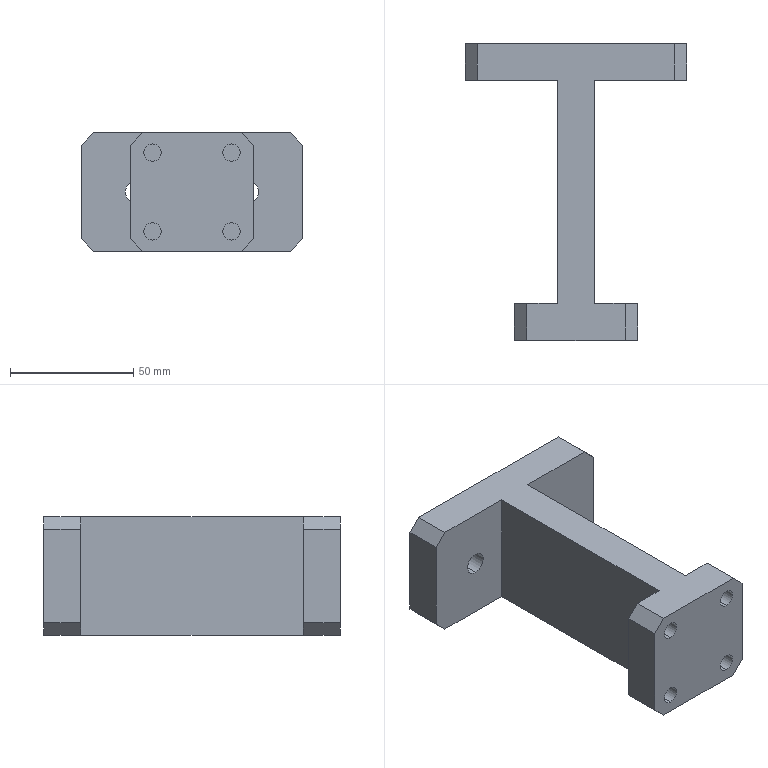Component | SolidWorks | TC020.05-06-2 | 1 solid | 34 faces | box 90 x 120.4 x 48 mm | volume 160170 mm3 | plane 22 | cylinder 12 | commonest cylinder face diameters 7 x8 9 x4 | material Q235A
STEP:
#1=CARTESIAN_POINT('',(4.901,3.307,0.7677));
#2=VERTEX_POINT('',#1);
#3=CARTESIAN_POINT('',(4.901,3.307,0.4921));
#4=VERTEX_POINT('',#3);
#5=CARTESIAN_POINT('',(4.901,3.307,0.6299));
#6=DIRECTION('',(0.,1.,0.));
#7=DIRECTION('',(0.,0.,1.));
#8=AXIS2_PLACEMENT_3D('',#5,#6,#7);
#9=CIRCLE('',#8,0.1378);
#10=EDGE_CURVE('',#2,#4,#9,.T.);
#11=ORIENTED_EDGE('',*,*,#10,.T.);
#12=CARTESIAN_POINT('',(4.901,2.717,0.4921));
#13=VERTEX_POINT('',#12);
#14=CARTESIAN_POINT('',(4.901,4.685,0.4921));
#15=DIRECTION('',(-0.,-1.,0.));
#16=VECTOR('',#15,39.37);
#17=LINE('',#14,#16);
#18=EDGE_CURVE('',#4,#13,#17,.T.);
#19=ORIENTED_EDGE('',*,*,#18,.T.);
#20=CARTESIAN_POINT('',(4.901,2.717,0.7677));
#21=VERTEX_POINT('',#20);
#22=CARTESIAN_POINT('',(4.901,2.717,0.6299));
#23=DIRECTION('',(0.,1.,0.));
#24=DIRECTION('',(0.,0.,-1.));
#25=AXIS2_PLACEMENT_3D('',#22,#23,#24);
#26=CIRCLE('',#25,0.1378);
#27=EDGE_CURVE('',#21,#13,#26,.T.);
#28=ORIENTED_EDGE('',*,*,#27,.F.);
#29=CARTESIAN_POINT('',(4.901,4.685,0.7677));
#30=DIRECTION('',(-0.,-1.,0.));
#31=VECTOR('',#30,39.37);
#32=LINE('',#29,#31);
#33=EDGE_CURVE('',#2,#21,#32,.T.);
#34=ORIENTED_EDGE('',*,*,#33,.F.);
#35=EDGE_LOOP('',(#11,#19,#28,#34));
#36=FACE_OUTER_BOUND('',#35,.T.);
#37=CARTESIAN_POINT('',(4.901,4.685,0.6299));
#38=DIRECTION('',(-0.,-1.,0.));
#39=DIRECTION('',(0.,0.,1.));
#40=AXIS2_PLACEMENT_3D('',#37,#38,#39);
#41=CYLINDRICAL_SURFACE('',#40,0.1378);
#42=ADVANCED_FACE('',(#36),#41,.F.);
#43=CARTESIAN_POINT('',(3.641,3.307,0.7677));
#44=VERTEX_POINT('',#43);
#45=CARTESIAN_POINT('',(3.641,3.307,0.4921));
#46=VERTEX_POINT('',#45);
#47=CARTESIAN_POINT('',(3.641,3.307,0.6299));
#48=DIRECTION('',(0.,1.,0.));
#49=DIRECTION('',(0.,0.,1.));
#50=AXIS2_PLACEMENT_3D('',#47,#48,#49);
#51=CIRCLE('',#50,0.1378);
#52=EDGE_CURVE('',#44,#46,#51,.T.);
#53=ORIENTED_EDGE('',*,*,#52,.T.);
#54=CARTESIAN_POINT('',(3.641,2.717,0.4921));
#55=VERTEX_POINT('',#54);
#56=CARTESIAN_POINT('',(3.641,4.685,0.4921));
#57=DIRECTION('',(-0.,-1.,0.));
#58=VECTOR('',#57,39.37);
#59=LINE('',#56,#58);
#60=EDGE_CURVE('',#46,#55,#59,.T.);
#61=ORIENTED_EDGE('',*,*,#60,.T.);
#62=CARTESIAN_POINT('',(3.641,2.717,0.7677));
#63=VERTEX_POINT('',#62);
#64=CARTESIAN_POINT('',(3.641,2.717,0.6299));
#65=DIRECTION('',(0.,1.,0.));
#66=DIRECTION('',(0.,0.,-1.));
#67=AXIS2_PLACEMENT_3D('',#64,#65,#66);
#68=CIRCLE('',#67,0.1378);
#69=EDGE_CURVE('',#63,#55,#68,.T.);
#70=ORIENTED_EDGE('',*,*,#69,.F.);
#71=CARTESIAN_POINT('',(3.641,4.685,0.7677));
#72=DIRECTION('',(-0.,-1.,0.));
#73=VECTOR('',#72,39.37);
#74=LINE('',#71,#73);
#75=EDGE_CURVE('',#44,#63,#74,.T.);
#76=ORIENTED_EDGE('',*,*,#75,.F.);
#77=EDGE_LOOP('',(#53,#61,#70,#76));
#78=FACE_OUTER_BOUND('',#77,.T.);
#79=CARTESIAN_POINT('',(3.641,4.685,0.6299));
#80=DIRECTION('',(-0.,-1.,0.));
#81=DIRECTION('',(0.,0.,1.));
#82=AXIS2_PLACEMENT_3D('',#79,#80,#81);
#83=CYLINDRICAL_SURFACE('',#82,0.1378);
#84=ADVANCED_FACE('',(#78),#83,.F.);
#85=CARTESIAN_POINT('',(4.901,3.307,-0.4921));
#86=VERTEX_POINT('',#85);
#87=CARTESIAN_POINT('',(4.901,3.307,-0.7677));
#88=VERTEX_POINT('',#87);
#89=CARTESIAN_POINT('',(4.901,3.307,-0.6299));
#90=DIRECTION('',(0.,1.,0.));
#91=DIRECTION('',(0.,0.,1.));
#92=AXIS2_PLACEMENT_3D('',#89,#90,#91);
#93=CIRCLE('',#92,0.1378);
#94=EDGE_CURVE('',#86,#88,#93,.T.);
#95=ORIENTED_EDGE('',*,*,#94,.T.);
#96=CARTESIAN_POINT('',(4.901,2.717,-0.7677));
#97=VERTEX_POINT('',#96);
#98=CARTESIAN_POINT('',(4.901,4.685,-0.7677));
#99=DIRECTION('',(-0.,-1.,0.));
#100=VECTOR('',#99,39.37);
#101=LINE('',#98,#100);
#102=EDGE_CURVE('',#88,#97,#101,.T.);
#103=ORIENTED_EDGE('',*,*,#102,.T.);
#104=CARTESIAN_POINT('',(4.901,2.717,-0.4921));
#105=VERTEX_POINT('',#104);
#106=CARTESIAN_POINT('',(4.901,2.717,-0.6299));
#107=DIRECTION('',(0.,1.,0.));
#108=DIRECTION('',(0.,0.,-1.));
#109=AXIS2_PLACEMENT_3D('',#106,#107,#108);
#110=CIRCLE('',#109,0.1378);
#111=EDGE_CURVE('',#105,#97,#110,.T.);
#112=ORIENTED_EDGE('',*,*,#111,.F.);
#113=CARTESIAN_POINT('',(4.901,4.685,-0.4921));
#114=DIRECTION('',(-0.,-1.,0.));
#115=VECTOR('',#114,39.37);
#116=LINE('',#113,#115);
#117=EDGE_CURVE('',#86,#105,#116,.T.);
#118=ORIENTED_EDGE('',*,*,#117,.F.);
#119=EDGE_LOOP('',(#95,#103,#112,#118));
#120=FACE_OUTER_BOUND('',#119,.T.);
#121=CARTESIAN_POINT('',(4.901,4.685,-0.6299));
#122=DIRECTION('',(-0.,-1.,0.));
#123=DIRECTION('',(0.,0.,1.));
#124=AXIS2_PLACEMENT_3D('',#121,#122,#123);
#125=CYLINDRICAL_SURFACE('',#124,0.1378);
#126=ADVANCED_FACE('',(#120),#125,.F.);
#127=CARTESIAN_POINT('',(3.641,3.307,-0.4921));
#128=VERTEX_POINT('',#127);
#129=CARTESIAN_POINT('',(3.641,3.307,-0.7677));
#130=VERTEX_POINT('',#129);
#131=CARTESIAN_POINT('',(3.641,3.307,-0.6299));
#132=DIRECTION('',(0.,1.,0.));
#133=DIRECTION('',(0.,0.,1.));
#134=AXIS2_PLACEMENT_3D('',#131,#132,#133);
#135=CIRCLE('',#134,0.1378);
#136=EDGE_CURVE('',#128,#130,#135,.T.);
#137=ORIENTED_EDGE('',*,*,#136,.T.);
#138=CARTESIAN_POINT('',(3.641,2.717,-0.7677));
#139=VERTEX_POINT('',#138);
#140=CARTESIAN_POINT('',(3.641,4.685,-0.7677));
#141=DIRECTION('',(-0.,-1.,0.));
#142=VECTOR('',#141,39.37);
#143=LINE('',#140,#142);
#144=EDGE_CURVE('',#130,#139,#143,.T.);
#145=ORIENTED_EDGE('',*,*,#144,.T.);
#146=CARTESIAN_POINT('',(3.641,2.717,-0.4921));
#147=VERTEX_POINT('',#146);
#148=CARTESIAN_POINT('',(3.641,2.717,-0.6299));
#149=DIRECTION('',(0.,1.,0.));
#150=DIRECTION('',(0.,0.,-1.));
#151=AXIS2_PLACEMENT_3D('',#148,#149,#150);
#152=CIRCLE('',#151,0.1378);
#153=EDGE_CURVE('',#147,#139,#152,.T.);
#154=ORIENTED_EDGE('',*,*,#153,.F.);
#155=CARTESIAN_POINT('',(3.641,4.685,-0.4921));
#156=DIRECTION('',(-0.,-1.,0.));
#157=VECTOR('',#156,39.37);
#158=LINE('',#155,#157);
#159=EDGE_CURVE('',#128,#147,#158,.T.);
#160=ORIENTED_EDGE('',*,*,#159,.F.);
#161=EDGE_LOOP('',(#137,#145,#154,#160));
#162=FACE_OUTER_BOUND('',#161,.T.);
#163=CARTESIAN_POINT('',(3.641,4.685,-0.6299));
#164=DIRECTION('',(-0.,-1.,0.));
#165=DIRECTION('',(0.,0.,1.));
#166=AXIS2_PLACEMENT_3D('',#163,#164,#165);
#167=CYLINDRICAL_SURFACE('',#166,0.1378);
#168=ADVANCED_FACE('',(#162),#167,.F.);
#169=CARTESIAN_POINT('',(3.386,6.866,-0.1772));
#170=VERTEX_POINT('',#169);
#171=CARTESIAN_POINT('',(3.386,6.866,0.1772));
#172=VERTEX_POINT('',#171);
#173=CARTESIAN_POINT('',(3.386,6.866,0.));
#174=DIRECTION('',(0.,-1.,0.));
#175=DIRECTION('',(-1.,0.,-0.));
#176=AXIS2_PLACEMENT_3D('',#173,#174,#175);
#177=CIRCLE('',#176,0.1772);
#178=EDGE_CURVE('',#170,#172,#177,.T.);
#179=ORIENTED_EDGE('',*,*,#178,.T.);
#180=CARTESIAN_POINT('',(3.386,7.457,0.1772));
#181=VERTEX_POINT('',#180);
#182=CARTESIAN_POINT('',(3.386,2.716,0.1772));
#183=DIRECTION('',(0.,1.,0.));
#184=VECTOR('',#183,39.37);
#185=LINE('',#182,#184);
#186=EDGE_CURVE('',#172,#181,#185,.T.);
#187=ORIENTED_EDGE('',*,*,#186,.T.);
#188=CARTESIAN_POINT('',(3.386,7.457,-0.1772));
#189=VERTEX_POINT('',#188);
#190=CARTESIAN_POINT('',(3.386,7.457,0.));
#191=DIRECTION('',(0.,1.,0.));
#192=DIRECTION('',(0.,0.,-1.));
#193=AXIS2_PLACEMENT_3D('',#190,#191,#192);
#194=CIRCLE('',#193,0.1772);
#195=EDGE_CURVE('',#181,#189,#194,.T.);
#196=ORIENTED_EDGE('',*,*,#195,.T.);
#197=CARTESIAN_POINT('',(3.386,2.716,-0.1772));
#198=DIRECTION('',(0.,1.,0.));
#199=VECTOR('',#198,39.37);
#200=LINE('',#197,#199);
#201=EDGE_CURVE('',#170,#189,#200,.T.);
#202=ORIENTED_EDGE('',*,*,#201,.F.);
#203=EDGE_LOOP('',(#179,#187,#196,#202));
#204=FACE_OUTER_BOUND('',#203,.T.);
#205=CARTESIAN_POINT('',(3.386,2.716,0.));
#206=DIRECTION('',(0.,1.,0.));
#207=DIRECTION('',(0.,0.,-1.));
#208=AXIS2_PLACEMENT_3D('',#205,#206,#207);
#209=CYLINDRICAL_SURFACE('',#208,0.1772);
#210=ADVANCED_FACE('',(#204),#209,.F.);
#211=CARTESIAN_POINT('',(5.157,6.866,-0.1772));
#212=VERTEX_POINT('',#211);
#213=CARTESIAN_POINT('',(5.157,6.866,0.1772));
#214=VERTEX_POINT('',#213);
#215=CARTESIAN_POINT('',(5.157,6.866,0.));
#216=DIRECTION('',(-0.,-1.,-0.));
#217=DIRECTION('',(-1.,0.,-0.));
#218=AXIS2_PLACEMENT_3D('',#215,#216,#217);
#219=CIRCLE('',#218,0.1772);
#220=EDGE_CURVE('',#212,#214,#219,.T.);
#221=ORIENTED_EDGE('',*,*,#220,.T.);
#222=CARTESIAN_POINT('',(5.157,7.457,0.1772));
#223=VERTEX_POINT('',#222);
#224=CARTESIAN_POINT('',(5.157,2.716,0.1772));
#225=DIRECTION('',(0.,1.,0.));
#226=VECTOR('',#225,39.37);
#227=LINE('',#224,#226);
#228=EDGE_CURVE('',#214,#223,#227,.T.);
#229=ORIENTED_EDGE('',*,*,#228,.T.);
#230=CARTESIAN_POINT('',(5.157,7.457,-0.1772));
#231=VERTEX_POINT('',#230);
#232=CARTESIAN_POINT('',(5.157,7.457,0.));
#233=DIRECTION('',(0.,1.,0.));
#234=DIRECTION('',(0.,0.,-1.));
#235=AXIS2_PLACEMENT_3D('',#232,#233,#234);
#236=CIRCLE('',#235,0.1772);
#237=EDGE_CURVE('',#223,#231,#236,.T.);
#238=ORIENTED_EDGE('',*,*,#237,.T.);
#239=CARTESIAN_POINT('',(5.157,2.716,-0.1772));
#240=DIRECTION('',(0.,1.,0.));
#241=VECTOR('',#240,39.37);
#242=LINE('',#239,#241);
#243=EDGE_CURVE('',#212,#231,#242,.T.);
#244=ORIENTED_EDGE('',*,*,#243,.F.);
#245=EDGE_LOOP('',(#221,#229,#238,#244));
#246=FACE_OUTER_BOUND('',#245,.T.);
#247=CARTESIAN_POINT('',(5.157,2.716,0.));
#248=DIRECTION('',(0.,1.,0.));
#249=DIRECTION('',(0.,0.,-1.));
#250=AXIS2_PLACEMENT_3D('',#247,#248,#249);
#251=CYLINDRICAL_SURFACE('',#250,0.1772);
#252=ADVANCED_FACE('',(#246),#251,.F.);
#253=CARTESIAN_POINT('',(3.484,2.717,0.9449));
#254=VERTEX_POINT('',#253);
#255=CARTESIAN_POINT('',(5.059,2.717,0.9449));
#256=VERTEX_POINT('',#255);
#257=CARTESIAN_POINT('',(3.287,2.717,0.9449));
#258=DIRECTION('',(1.,-0.,0.));
#259=VECTOR('',#258,39.37);
#260=LINE('',#257,#259);
#261=EDGE_CURVE('',#254,#256,#260,.T.);
#262=ORIENTED_EDGE('',*,*,#261,.F.);
#263=CARTESIAN_POINT('',(3.287,2.717,0.748));
#264=VERTEX_POINT('',#263);
#265=CARTESIAN_POINT('',(3.484,2.717,0.9449));
#266=DIRECTION('',(-0.7071,0.,-0.7071));
#267=VECTOR('',#266,39.37);
#268=LINE('',#265,#267);
#269=EDGE_CURVE('',#254,#264,#268,.T.);
#270=ORIENTED_EDGE('',*,*,#269,.T.);
#271=CARTESIAN_POINT('',(3.287,2.717,-0.748));
#272=VERTEX_POINT('',#271);
#273=CARTESIAN_POINT('',(3.287,2.717,0.9449));
#274=DIRECTION('',(0.,0.,-1.));
#275=VECTOR('',#274,39.37);
#276=LINE('',#273,#275);
#277=EDGE_CURVE('',#264,#272,#276,.T.);
#278=ORIENTED_EDGE('',*,*,#277,.T.);
#279=CARTESIAN_POINT('',(3.484,2.717,-0.9449));
#280=VERTEX_POINT('',#279);
#281=CARTESIAN_POINT('',(3.287,2.717,-0.748));
#282=DIRECTION('',(0.7071,-0.,-0.7071));
#283=VECTOR('',#282,39.37);
#284=LINE('',#281,#283);
#285=EDGE_CURVE('',#272,#280,#284,.T.);
#286=ORIENTED_EDGE('',*,*,#285,.T.);
#287=CARTESIAN_POINT('',(5.059,2.717,-0.9449));
#288=VERTEX_POINT('',#287);
#289=CARTESIAN_POINT('',(3.287,2.717,-0.9449));
#290=DIRECTION('',(1.,-0.,0.));
#291=VECTOR('',#290,39.37);
#292=LINE('',#289,#291);
#293=EDGE_CURVE('',#280,#288,#292,.T.);
#294=ORIENTED_EDGE('',*,*,#293,.T.);
#295=CARTESIAN_POINT('',(5.256,2.717,-0.748));
#296=VERTEX_POINT('',#295);
#297=CARTESIAN_POINT('',(5.256,2.717,-0.748));
#298=DIRECTION('',(0.7071,-0.,0.7071));
#299=VECTOR('',#298,39.37);
#300=LINE('',#297,#299);
#301=EDGE_CURVE('',#288,#296,#300,.T.);
#302=ORIENTED_EDGE('',*,*,#301,.T.);
#303=CARTESIAN_POINT('',(5.256,2.717,0.748));
#304=VERTEX_POINT('',#303);
#305=CARTESIAN_POINT('',(5.256,2.717,0.9449));
#306=DIRECTION('',(0.,0.,-1.));
#307=VECTOR('',#306,39.37);
#308=LINE('',#305,#307);
#309=EDGE_CURVE('',#304,#296,#308,.T.);
#310=ORIENTED_EDGE('',*,*,#309,.F.);
#311=CARTESIAN_POINT('',(5.059,2.717,0.9449));
#312=DIRECTION('',(-0.7071,0.,0.7071));
#313=VECTOR('',#312,39.37);
#314=LINE('',#311,#313);
#315=EDGE_CURVE('',#304,#256,#314,.T.);
#316=ORIENTED_EDGE('',*,*,#315,.T.);
#317=EDGE_LOOP('',(#262,#270,#278,#286,#294,#302,#310,#316));
#318=FACE_OUTER_BOUND('',#317,.T.);
#319=ORIENTED_EDGE('',*,*,#153,.T.);
#320=CARTESIAN_POINT('',(3.641,2.717,-0.6299));
#321=DIRECTION('',(0.,1.,0.));
#322=DIRECTION('',(0.,0.,-1.));
#323=AXIS2_PLACEMENT_3D('',#320,#321,#322);
#324=CIRCLE('',#323,0.1378);
#325=EDGE_CURVE('',#139,#147,#324,.T.);
#326=ORIENTED_EDGE('',*,*,#325,.T.);
#327=EDGE_LOOP('',(#319,#326));
#328=FACE_BOUND('',#327,.T.);
#329=ORIENTED_EDGE('',*,*,#111,.T.);
#330=CARTESIAN_POINT('',(4.901,2.717,-0.6299));
#331=DIRECTION('',(0.,1.,0.));
#332=DIRECTION('',(0.,0.,-1.));
#333=AXIS2_PLACEMENT_3D('',#330,#331,#332);
#334=CIRCLE('',#333,0.1378);
#335=EDGE_CURVE('',#97,#105,#334,.T.);
#336=ORIENTED_EDGE('',*,*,#335,.T.);
#337=EDGE_LOOP('',(#329,#336));
#338=FACE_BOUND('',#337,.T.);
#339=ORIENTED_EDGE('',*,*,#69,.T.);
#340=CARTESIAN_POINT('',(3.641,2.717,0.6299));
#341=DIRECTION('',(0.,1.,0.));
#342=DIRECTION('',(0.,0.,-1.));
#343=AXIS2_PLACEMENT_3D('',#340,#341,#342);
#344=CIRCLE('',#343,0.1378);
#345=EDGE_CURVE('',#55,#63,#344,.T.);
#346=ORIENTED_EDGE('',*,*,#345,.T.);
#347=EDGE_LOOP('',(#339,#346));
#348=FACE_BOUND('',#347,.T.);
#349=ORIENTED_EDGE('',*,*,#27,.T.);
#350=CARTESIAN_POINT('',(4.901,2.717,0.6299));
#351=DIRECTION('',(0.,1.,0.));
#352=DIRECTION('',(0.,0.,-1.));
#353=AXIS2_PLACEMENT_3D('',#350,#351,#352);
#354=CIRCLE('',#353,0.1378);
#355=EDGE_CURVE('',#13,#21,#354,.T.);
#356=ORIENTED_EDGE('',*,*,#355,.T.);
#357=EDGE_LOOP('',(#349,#356));
#358=FACE_BOUND('',#357,.T.);
#359=CARTESIAN_POINT('',(3.287,2.717,0.9449));
#360=DIRECTION('',(0.,1.,0.));
#361=DIRECTION('',(0.,0.,-1.));
#362=AXIS2_PLACEMENT_3D('',#359,#360,#361);
#363=PLANE('',#362);
#364=ADVANCED_FACE('',(#318,#328,#338,#348,#358),#363,.F.);
#365=CARTESIAN_POINT('',(5.059,3.307,0.9449));
#366=VERTEX_POINT('',#365);
#367=CARTESIAN_POINT('',(4.567,3.307,0.9449));
#368=VERTEX_POINT('',#367);
#369=CARTESIAN_POINT('',(4.567,3.307,0.9449));
#370=DIRECTION('',(-1.,0.,-0.));
#371=VECTOR('',#370,39.37);
#372=LINE('',#369,#371);
#373=EDGE_CURVE('',#366,#368,#372,.T.);
#374=ORIENTED_EDGE('',*,*,#373,.F.);
#375=CARTESIAN_POINT('',(5.256,3.307,0.748));
#376=VERTEX_POINT('',#375);
#377=CARTESIAN_POINT('',(5.059,3.307,0.9449));
#378=DIRECTION('',(0.7071,-0.,-0.7071));
#379=VECTOR('',#378,39.37);
#380=LINE('',#377,#379);
#381=EDGE_CURVE('',#366,#376,#380,.T.);
#382=ORIENTED_EDGE('',*,*,#381,.T.);
#383=CARTESIAN_POINT('',(5.256,3.307,-0.748));
#384=VERTEX_POINT('',#383);
#385=CARTESIAN_POINT('',(5.256,3.307,0.9449));
#386=DIRECTION('',(0.,0.,-1.));
#387=VECTOR('',#386,39.37);
#388=LINE('',#385,#387);
#389=EDGE_CURVE('',#376,#384,#388,.T.);
#390=ORIENTED_EDGE('',*,*,#389,.T.);
#391=CARTESIAN_POINT('',(5.059,3.307,-0.9449));
#392=VERTEX_POINT('',#391);
#393=CARTESIAN_POINT('',(5.256,3.307,-0.748));
#394=DIRECTION('',(-0.7071,0.,-0.7071));
#395=VECTOR('',#394,39.37);
#396=LINE('',#393,#395);
#397=EDGE_CURVE('',#384,#392,#396,.T.);
#398=ORIENTED_EDGE('',*,*,#397,.T.);
#399=CARTESIAN_POINT('',(4.567,3.307,-0.9449));
#400=VERTEX_POINT('',#399);
#401=CARTESIAN_POINT('',(4.567,3.307,-0.9449));
#402=DIRECTION('',(-1.,0.,-0.));
#403=VECTOR('',#402,39.37);
#404=LINE('',#401,#403);
#405=EDGE_CURVE('',#392,#400,#404,.T.);
#406=ORIENTED_EDGE('',*,*,#405,.T.);
#407=CARTESIAN_POINT('',(4.567,3.307,0.9449));
#408=DIRECTION('',(0.,0.,-1.));
#409=VECTOR('',#408,39.37);
#410=LINE('',#407,#409);
#411=EDGE_CURVE('',#368,#400,#410,.T.);
#412=ORIENTED_EDGE('',*,*,#411,.F.);
#413=EDGE_LOOP('',(#374,#382,#390,#398,#406,#412));
#414=FACE_OUTER_BOUND('',#413,.T.);
#415=ORIENTED_EDGE('',*,*,#94,.F.);
#416=CARTESIAN_POINT('',(4.901,3.307,-0.6299));
#417=DIRECTION('',(0.,1.,0.));
#418=DIRECTION('',(0.,0.,1.));
#419=AXIS2_PLACEMENT_3D('',#416,#417,#418);
#420=CIRCLE('',#419,0.1378);
#421=EDGE_CURVE('',#88,#86,#420,.T.);
#422=ORIENTED_EDGE('',*,*,#421,.F.);
#423=EDGE_LOOP('',(#415,#422));
#424=FACE_BOUND('',#423,.T.);
#425=ORIENTED_EDGE('',*,*,#10,.F.);
#426=CARTESIAN_POINT('',(4.901,3.307,0.6299));
#427=DIRECTION('',(0.,1.,0.));
#428=DIRECTION('',(0.,0.,1.));
#429=AXIS2_PLACEMENT_3D('',#426,#427,#428);
#430=CIRCLE('',#429,0.1378);
#431=EDGE_CURVE('',#4,#2,#430,.T.);
#432=ORIENTED_EDGE('',*,*,#431,.F.);
#433=EDGE_LOOP('',(#425,#432));
#434=FACE_BOUND('',#433,.T.);
#435=CARTESIAN_POINT('',(4.567,3.307,0.9449));
#436=DIRECTION('',(-0.,-1.,-0.));
#437=DIRECTION('',(-0.,0.,1.));
#438=AXIS2_PLACEMENT_3D('',#435,#436,#437);
#439=PLANE('',#438);
#440=ADVANCED_FACE('',(#414,#424,#434),#439,.F.);
#441=CARTESIAN_POINT('',(3.287,3.307,0.748));
#442=VERTEX_POINT('',#441);
#443=CARTESIAN_POINT('',(3.287,3.307,-0.748));
#444=VERTEX_POINT('',#443);
#445=CARTESIAN_POINT('',(3.287,3.307,0.9449));
#446=DIRECTION('',(0.,0.,-1.));
#447=VECTOR('',#446,39.37);
#448=LINE('',#445,#447);
#449=EDGE_CURVE('',#442,#444,#448,.T.);
#450=ORIENTED_EDGE('',*,*,#449,.F.);
#451=CARTESIAN_POINT('',(3.484,3.307,0.9449));
#452=VERTEX_POINT('',#451);
#453=CARTESIAN_POINT('',(3.484,3.307,0.9449));
#454=DIRECTION('',(0.7071,-0.,0.7071));
#455=VECTOR('',#454,39.37);
#456=LINE('',#453,#455);
#457=EDGE_CURVE('',#442,#452,#456,.T.);
#458=ORIENTED_EDGE('',*,*,#457,.T.);
#459=CARTESIAN_POINT('',(3.976,3.307,0.9449));
#460=VERTEX_POINT('',#459);
#461=CARTESIAN_POINT('',(3.976,3.307,0.9449));
#462=DIRECTION('',(-1.,0.,-0.));
#463=VECTOR('',#462,39.37);
#464=LINE('',#461,#463);
#465=EDGE_CURVE('',#460,#452,#464,.T.);
#466=ORIENTED_EDGE('',*,*,#465,.F.);
#467=CARTESIAN_POINT('',(3.976,3.307,-0.9449));
#468=VERTEX_POINT('',#467);
#469=CARTESIAN_POINT('',(3.976,3.307,0.9449));
#470=DIRECTION('',(0.,0.,-1.));
#471=VECTOR('',#470,39.37);
#472=LINE('',#469,#471);
#473=EDGE_CURVE('',#460,#468,#472,.T.);
#474=ORIENTED_EDGE('',*,*,#473,.T.);
#475=CARTESIAN_POINT('',(3.484,3.307,-0.9449));
#476=VERTEX_POINT('',#475);
#477=CARTESIAN_POINT('',(3.976,3.307,-0.9449));
#478=DIRECTION('',(-1.,0.,-0.));
#479=VECTOR('',#478,39.37);
#480=LINE('',#477,#479);
#481=EDGE_CURVE('',#468,#476,#480,.T.);
#482=ORIENTED_EDGE('',*,*,#481,.T.);
#483=CARTESIAN_POINT('',(3.287,3.307,-0.748));
#484=DIRECTION('',(-0.7071,0.,0.7071));
#485=VECTOR('',#484,39.37);
#486=LINE('',#483,#485);
#487=EDGE_CURVE('',#476,#444,#486,.T.);
#488=ORIENTED_EDGE('',*,*,#487,.T.);
#489=EDGE_LOOP('',(#450,#458,#466,#474,#482,#488));
#490=FACE_OUTER_BOUND('',#489,.T.);
#491=ORIENTED_EDGE('',*,*,#136,.F.);
#492=CARTESIAN_POINT('',(3.641,3.307,-0.6299));
#493=DIRECTION('',(0.,1.,0.));
#494=DIRECTION('',(0.,0.,1.));
#495=AXIS2_PLACEMENT_3D('',#492,#493,#494);
#496=CIRCLE('',#495,0.1378);
#497=EDGE_CURVE('',#130,#128,#496,.T.);
#498=ORIENTED_EDGE('',*,*,#497,.F.);
#499=EDGE_LOOP('',(#491,#498));
#500=FACE_BOUND('',#499,.T.);
#501=ORIENTED_EDGE('',*,*,#52,.F.);
#502=CARTESIAN_POINT('',(3.641,3.307,0.6299));
#503=DIRECTION('',(0.,1.,0.));
#504=DIRECTION('',(0.,0.,1.));
#505=AXIS2_PLACEMENT_3D('',#502,#503,#504);
#506=CIRCLE('',#505,0.1378);
#507=EDGE_CURVE('',#46,#44,#506,.T.);
#508=ORIENTED_EDGE('',*,*,#507,.F.);
#509=EDGE_LOOP('',(#501,#508));
#510=FACE_BOUND('',#509,.T.);
#511=CARTESIAN_POINT('',(3.976,3.307,0.9449));
#512=DIRECTION('',(-0.,-1.,-0.));
#513=DIRECTION('',(-0.,0.,1.));
#514=AXIS2_PLACEMENT_3D('',#511,#512,#513);
#515=PLANE('',#514);
#516=ADVANCED_FACE('',(#490,#500,#510),#515,.F.);
#517=ORIENTED_EDGE('',*,*,#178,.F.);
#518=CARTESIAN_POINT('',(3.386,6.866,0.));
#519=DIRECTION('',(0.,-1.,0.));
#520=DIRECTION('',(-1.,0.,-0.));
#521=AXIS2_PLACEMENT_3D('',#518,#519,#520);
#522=CIRCLE('',#521,0.1772);
#523=EDGE_CURVE('',#172,#170,#522,.T.);
#524=ORIENTED_EDGE('',*,*,#523,.F.);
#525=EDGE_LOOP('',(#517,#524));
#526=FACE_BOUND('',#525,.T.);
#527=CARTESIAN_POINT('',(2.697,6.866,0.9449));
#528=VERTEX_POINT('',#527);
#529=CARTESIAN_POINT('',(3.976,6.866,0.9449));
#530=VERTEX_POINT('',#529);
#531=CARTESIAN_POINT('',(2.5,6.866,0.9449));
#532=DIRECTION('',(1.,0.,0.));
#533=VECTOR('',#532,39.37);
#534=LINE('',#531,#533);
#535=EDGE_CURVE('',#528,#530,#534,.T.);
#536=ORIENTED_EDGE('',*,*,#535,.F.);
#537=CARTESIAN_POINT('',(2.5,6.866,0.748));
#538=VERTEX_POINT('',#537);
#539=CARTESIAN_POINT('',(2.697,6.866,0.9449));
#540=DIRECTION('',(-0.7071,-0.,-0.7071));
#541=VECTOR('',#540,39.37);
#542=LINE('',#539,#541);
#543=EDGE_CURVE('',#528,#538,#542,.T.);
#544=ORIENTED_EDGE('',*,*,#543,.T.);
#545=CARTESIAN_POINT('',(2.5,6.866,-0.748));
#546=VERTEX_POINT('',#545);
#547=CARTESIAN_POINT('',(2.5,6.866,0.9449));
#548=DIRECTION('',(0.,0.,-1.));
#549=VECTOR('',#548,39.37);
#550=LINE('',#547,#549);
#551=EDGE_CURVE('',#538,#546,#550,.T.);
#552=ORIENTED_EDGE('',*,*,#551,.T.);
#553=CARTESIAN_POINT('',(2.697,6.866,-0.9449));
#554=VERTEX_POINT('',#553);
#555=CARTESIAN_POINT('',(2.5,6.866,-0.748));
#556=DIRECTION('',(0.7071,0.,-0.7071));
#557=VECTOR('',#556,39.37);
#558=LINE('',#555,#557);
#559=EDGE_CURVE('',#546,#554,#558,.T.);
#560=ORIENTED_EDGE('',*,*,#559,.T.);
#561=CARTESIAN_POINT('',(3.976,6.866,-0.9449));
#562=VERTEX_POINT('',#561);
#563=CARTESIAN_POINT('',(2.5,6.866,-0.9449));
#564=DIRECTION('',(1.,0.,0.));
#565=VECTOR('',#564,39.37);
#566=LINE('',#563,#565);
#567=EDGE_CURVE('',#554,#562,#566,.T.);
#568=ORIENTED_EDGE('',*,*,#567,.T.);
#569=CARTESIAN_POINT('',(3.976,6.866,0.9449));
#570=DIRECTION('',(0.,0.,-1.));
#571=VECTOR('',#570,39.37);
#572=LINE('',#569,#571);
#573=EDGE_CURVE('',#530,#562,#572,.T.);
#574=ORIENTED_EDGE('',*,*,#573,.F.);
#575=EDGE_LOOP('',(#536,#544,#552,#560,#568,#574));
#576=FACE_OUTER_BOUND('',#575,.T.);
#577=CARTESIAN_POINT('',(2.5,6.866,0.9449));
#578=DIRECTION('',(-0.,1.,-0.));
#579=DIRECTION('',(-1.,-0.,-0.));
#580=AXIS2_PLACEMENT_3D('',#577,#578,#579);
#581=PLANE('',#580);
#582=ADVANCED_FACE('',(#526,#576),#581,.F.);
#583=CARTESIAN_POINT('',(3.976,6.866,-0.9449));
#584=DIRECTION('',(-0.,-1.,0.));
#585=VECTOR('',#584,39.37);
#586=LINE('',#583,#585);
#587=EDGE_CURVE('',#562,#468,#586,.T.);
#588=ORIENTED_EDGE('',*,*,#587,.T.);
#589=ORIENTED_EDGE('',*,*,#473,.F.);
#590=CARTESIAN_POINT('',(3.976,6.866,0.9449));
#591=DIRECTION('',(-0.,-1.,0.));
#592=VECTOR('',#591,39.37);
#593=LINE('',#590,#592);
#594=EDGE_CURVE('',#530,#460,#593,.T.);
#595=ORIENTED_EDGE('',*,*,#594,.F.);
#596=ORIENTED_EDGE('',*,*,#573,.T.);
#597=EDGE_LOOP('',(#588,#589,#595,#596));
#598=FACE_OUTER_BOUND('',#597,.T.);
#599=CARTESIAN_POINT('',(3.976,6.866,0.9449));
#600=DIRECTION('',(1.,-0.,0.));
#601=DIRECTION('',(-0.,0.,1.));
#602=AXIS2_PLACEMENT_3D('',#599,#600,#601);
#603=PLANE('',#602);
#604=ADVANCED_FACE('',(#598),#603,.F.);
#605=ORIENTED_EDGE('',*,*,#277,.F.);
#606=CARTESIAN_POINT('',(3.287,3.307,0.748));
#607=DIRECTION('',(0.,1.,0.));
#608=VECTOR('',#607,39.37);
#609=LINE('',#606,#608);
#610=EDGE_CURVE('',#264,#442,#609,.T.);
#611=ORIENTED_EDGE('',*,*,#610,.T.);
#612=ORIENTED_EDGE('',*,*,#449,.T.);
#613=CARTESIAN_POINT('',(3.287,2.717,-0.748));
#614=DIRECTION('',(-0.,-1.,0.));
#615=VECTOR('',#614,39.37);
#616=LINE('',#613,#615);
#617=EDGE_CURVE('',#444,#272,#616,.T.);
#618=ORIENTED_EDGE('',*,*,#617,.T.);
#619=EDGE_LOOP('',(#605,#611,#612,#618));
#620=FACE_OUTER_BOUND('',#619,.T.);
#621=CARTESIAN_POINT('',(3.287,3.307,0.9449));
#622=DIRECTION('',(1.,-0.,0.));
#623=DIRECTION('',(-0.,0.,1.));
#624=AXIS2_PLACEMENT_3D('',#621,#622,#623);
#625=PLANE('',#624);
#626=ADVANCED_FACE('',(#620),#625,.F.);
#627=ORIENTED_EDGE('',*,*,#389,.F.);
#628=CARTESIAN_POINT('',(5.256,3.307,0.748));
#629=DIRECTION('',(-0.,-1.,0.));
#630=VECTOR('',#629,39.37);
#631=LINE('',#628,#630);
#632=EDGE_CURVE('',#376,#304,#631,.T.);
#633=ORIENTED_EDGE('',*,*,#632,.T.);
#634=ORIENTED_EDGE('',*,*,#309,.T.);
#635=CARTESIAN_POINT('',(5.256,3.307,-0.748));
#636=DIRECTION('',(0.,1.,0.));
#637=VECTOR('',#636,39.37);
#638=LINE('',#635,#637);
#639=EDGE_CURVE('',#296,#384,#638,.T.);
#640=ORIENTED_EDGE('',*,*,#639,.T.);
#641=EDGE_LOOP('',(#627,#633,#634,#640));
#642=FACE_OUTER_BOUND('',#641,.T.);
#643=CARTESIAN_POINT('',(5.256,3.307,0.9449));
#644=DIRECTION('',(-1.,0.,-0.));
#645=DIRECTION('',(0.,0.,-1.));
#646=AXIS2_PLACEMENT_3D('',#643,#644,#645);
#647=PLANE('',#646);
#648=ADVANCED_FACE('',(#642),#647,.F.);
#649=CARTESIAN_POINT('',(4.567,6.866,-0.9449));
#650=VERTEX_POINT('',#649);
#651=CARTESIAN_POINT('',(4.567,6.866,-0.9449));
#652=DIRECTION('',(0.,1.,0.));
#653=VECTOR('',#652,39.37);
#654=LINE('',#651,#653);
#655=EDGE_CURVE('',#400,#650,#654,.T.);
#656=ORIENTED_EDGE('',*,*,#655,.T.);
#657=CARTESIAN_POINT('',(4.567,6.866,0.9449));
#658=VERTEX_POINT('',#657);
#659=CARTESIAN_POINT('',(4.567,6.866,0.9449));
#660=DIRECTION('',(0.,0.,-1.));
#661=VECTOR('',#660,39.37);
#662=LINE('',#659,#661);
#663=EDGE_CURVE('',#658,#650,#662,.T.);
#664=ORIENTED_EDGE('',*,*,#663,.F.);
#665=CARTESIAN_POINT('',(4.567,6.866,0.9449));
#666=DIRECTION('',(0.,1.,0.));
#667=VECTOR('',#666,39.37);
#668=LINE('',#665,#667);
#669=EDGE_CURVE('',#368,#658,#668,.T.);
#670=ORIENTED_EDGE('',*,*,#669,.F.);
#671=ORIENTED_EDGE('',*,*,#411,.T.);
#672=EDGE_LOOP('',(#656,#664,#670,#671));
#673=FACE_OUTER_BOUND('',#672,.T.);
#674=CARTESIAN_POINT('',(4.567,6.866,0.9449));
#675=DIRECTION('',(-1.,0.,-0.));
#676=DIRECTION('',(0.,0.,-1.));
#677=AXIS2_PLACEMENT_3D('',#674,#675,#676);
#678=PLANE('',#677);
#679=ADVANCED_FACE('',(#673),#678,.F.);
#680=ORIENTED_EDGE('',*,*,#220,.F.);
#681=CARTESIAN_POINT('',(5.157,6.866,0.));
#682=DIRECTION('',(-0.,-1.,-0.));
#683=DIRECTION('',(-1.,0.,-0.));
#684=AXIS2_PLACEMENT_3D('',#681,#682,#683);
#685=CIRCLE('',#684,0.1772);
#686=EDGE_CURVE('',#214,#212,#685,.T.);
#687=ORIENTED_EDGE('',*,*,#686,.F.);
#688=EDGE_LOOP('',(#680,#687));
#689=FACE_BOUND('',#688,.T.);
#690=CARTESIAN_POINT('',(6.043,6.866,0.748));
#691=VERTEX_POINT('',#690);
#692=CARTESIAN_POINT('',(6.043,6.866,-0.748));
#693=VERTEX_POINT('',#692);
#694=CARTESIAN_POINT('',(6.043,6.866,0.9449));
#695=DIRECTION('',(0.,0.,-1.));
#696=VECTOR('',#695,39.37);
#697=LINE('',#694,#696);
#698=EDGE_CURVE('',#691,#693,#697,.T.);
#699=ORIENTED_EDGE('',*,*,#698,.F.);
#700=CARTESIAN_POINT('',(5.846,6.866,0.9449));
#701=VERTEX_POINT('',#700);
#702=CARTESIAN_POINT('',(5.846,6.866,0.9449));
#703=DIRECTION('',(-0.7071,0.,0.7071));
#704=VECTOR('',#703,39.37);
#705=LINE('',#702,#704);
#706=EDGE_CURVE('',#691,#701,#705,.T.);
#707=ORIENTED_EDGE('',*,*,#706,.T.);
#708=CARTESIAN_POINT('',(6.043,6.866,0.9449));
#709=DIRECTION('',(1.,-0.,0.));
#710=VECTOR('',#709,39.37);
#711=LINE('',#708,#710);
#712=EDGE_CURVE('',#658,#701,#711,.T.);
#713=ORIENTED_EDGE('',*,*,#712,.F.);
#714=ORIENTED_EDGE('',*,*,#663,.T.);
#715=CARTESIAN_POINT('',(5.846,6.866,-0.9449));
#716=VERTEX_POINT('',#715);
#717=CARTESIAN_POINT('',(6.043,6.866,-0.9449));
#718=DIRECTION('',(1.,-0.,0.));
#719=VECTOR('',#718,39.37);
#720=LINE('',#717,#719);
#721=EDGE_CURVE('',#650,#716,#720,.T.);
#722=ORIENTED_EDGE('',*,*,#721,.T.);
#723=CARTESIAN_POINT('',(6.043,6.866,-0.748));
#724=DIRECTION('',(0.7071,-0.,0.7071));
#725=VECTOR('',#724,39.37);
#726=LINE('',#723,#725);
#727=EDGE_CURVE('',#716,#693,#726,.T.);
#728=ORIENTED_EDGE('',*,*,#727,.T.);
#729=EDGE_LOOP('',(#699,#707,#713,#714,#722,#728));
#730=FACE_OUTER_BOUND('',#729,.T.);
#731=CARTESIAN_POINT('',(6.043,6.866,0.9449));
#732=DIRECTION('',(0.,1.,0.));
#733=DIRECTION('',(-1.,0.,-0.));
#734=AXIS2_PLACEMENT_3D('',#731,#732,#733);
#735=PLANE('',#734);
#736=ADVANCED_FACE('',(#689,#730),#735,.F.);
#737=CARTESIAN_POINT('',(6.043,7.457,0.748));
#738=VERTEX_POINT('',#737);
#739=CARTESIAN_POINT('',(6.043,7.457,-0.748));
#740=VERTEX_POINT('',#739);
#741=CARTESIAN_POINT('',(6.043,7.457,0.9449));
#742=DIRECTION('',(0.,0.,-1.));
#743=VECTOR('',#742,39.37);
#744=LINE('',#741,#743);
#745=EDGE_CURVE('',#738,#740,#744,.T.);
#746=ORIENTED_EDGE('',*,*,#745,.F.);
#747=CARTESIAN_POINT('',(6.043,7.457,0.748));
#748=DIRECTION('',(-0.,-1.,0.));
#749=VECTOR('',#748,39.37);
#750=LINE('',#747,#749);
#751=EDGE_CURVE('',#738,#691,#750,.T.);
#752=ORIENTED_EDGE('',*,*,#751,.T.);
#753=ORIENTED_EDGE('',*,*,#698,.T.);
#754=CARTESIAN_POINT('',(6.043,7.457,-0.748));
#755=DIRECTION('',(0.,1.,0.));
#756=VECTOR('',#755,39.37);
#757=LINE('',#754,#756);
#758=EDGE_CURVE('',#693,#740,#757,.T.);
#759=ORIENTED_EDGE('',*,*,#758,.T.);
#760=EDGE_LOOP('',(#746,#752,#753,#759));
#761=FACE_OUTER_BOUND('',#760,.T.);
#762=CARTESIAN_POINT('',(6.043,7.457,0.9449));
#763=DIRECTION('',(-1.,0.,-0.));
#764=DIRECTION('',(0.,0.,-1.));
#765=AXIS2_PLACEMENT_3D('',#762,#763,#764);
#766=PLANE('',#765);
#767=ADVANCED_FACE('',(#761),#766,.F.);
#768=CARTESIAN_POINT('',(3.386,7.457,0.));
#769=DIRECTION('',(0.,1.,0.));
#770=DIRECTION('',(0.,0.,-1.));
#771=AXIS2_PLACEMENT_3D('',#768,#769,#770);
#772=CIRCLE('',#771,0.1772);
#773=EDGE_CURVE('',#189,#181,#772,.T.);
#774=ORIENTED_EDGE('',*,*,#773,.F.);
#775=ORIENTED_EDGE('',*,*,#195,.F.);
#776=EDGE_LOOP('',(#774,#775));
#777=FACE_BOUND('',#776,.T.);
#778=CARTESIAN_POINT('',(5.157,7.457,0.));
#779=DIRECTION('',(0.,1.,0.));
#780=DIRECTION('',(0.,0.,-1.));
#781=AXIS2_PLACEMENT_3D('',#778,#779,#780);
#782=CIRCLE('',#781,0.1772);
#783=EDGE_CURVE('',#231,#223,#782,.T.);
#784=ORIENTED_EDGE('',*,*,#783,.F.);
#785=ORIENTED_EDGE('',*,*,#237,.F.);
#786=EDGE_LOOP('',(#784,#785));
#787=FACE_BOUND('',#786,.T.);
#788=CARTESIAN_POINT('',(5.846,7.457,0.9449));
#789=VERTEX_POINT('',#788);
#790=CARTESIAN_POINT('',(2.697,7.457,0.9449));
#791=VERTEX_POINT('',#790);
#792=CARTESIAN_POINT('',(6.043,7.457,0.9449));
#793=DIRECTION('',(-1.,0.,-0.));
#794=VECTOR('',#793,39.37);
#795=LINE('',#792,#794);
#796=EDGE_CURVE('',#789,#791,#795,.T.);
#797=ORIENTED_EDGE('',*,*,#796,.F.);
#798=CARTESIAN_POINT('',(5.846,7.457,0.9449));
#799=DIRECTION('',(0.7071,-0.,-0.7071));
#800=VECTOR('',#799,39.37);
#801=LINE('',#798,#800);
#802=EDGE_CURVE('',#789,#738,#801,.T.);
#803=ORIENTED_EDGE('',*,*,#802,.T.);
#804=ORIENTED_EDGE('',*,*,#745,.T.);
#805=CARTESIAN_POINT('',(5.846,7.457,-0.9449));
#806=VERTEX_POINT('',#805);
#807=CARTESIAN_POINT('',(6.043,7.457,-0.748));
#808=DIRECTION('',(-0.7071,0.,-0.7071));
#809=VECTOR('',#808,39.37);
#810=LINE('',#807,#809);
#811=EDGE_CURVE('',#740,#806,#810,.T.);
#812=ORIENTED_EDGE('',*,*,#811,.T.);
#813=CARTESIAN_POINT('',(2.697,7.457,-0.9449));
#814=VERTEX_POINT('',#813);
#815=CARTESIAN_POINT('',(6.043,7.457,-0.9449));
#816=DIRECTION('',(-1.,0.,-0.));
#817=VECTOR('',#816,39.37);
#818=LINE('',#815,#817);
#819=EDGE_CURVE('',#806,#814,#818,.T.);
#820=ORIENTED_EDGE('',*,*,#819,.T.);
#821=CARTESIAN_POINT('',(2.5,7.457,-0.748));
#822=VERTEX_POINT('',#821);
#823=CARTESIAN_POINT('',(2.5,7.457,-0.748));
#824=DIRECTION('',(-0.7071,0.,0.7071));
#825=VECTOR('',#824,39.37);
#826=LINE('',#823,#825);
#827=EDGE_CURVE('',#814,#822,#826,.T.);
#828=ORIENTED_EDGE('',*,*,#827,.T.);
#829=CARTESIAN_POINT('',(2.5,7.457,0.748));
#830=VERTEX_POINT('',#829);
#831=CARTESIAN_POINT('',(2.5,7.457,0.9449));
#832=DIRECTION('',(0.,0.,-1.));
#833=VECTOR('',#832,39.37);
#834=LINE('',#831,#833);
#835=EDGE_CURVE('',#830,#822,#834,.T.);
#836=ORIENTED_EDGE('',*,*,#835,.F.);
#837=CARTESIAN_POINT('',(2.697,7.457,0.9449));
#838=DIRECTION('',(0.7071,-0.,0.7071));
#839=VECTOR('',#838,39.37);
#840=LINE('',#837,#839);
#841=EDGE_CURVE('',#830,#791,#840,.T.);
#842=ORIENTED_EDGE('',*,*,#841,.T.);
#843=EDGE_LOOP('',(#797,#803,#804,#812,#820,#828,#836,#842));
#844=FACE_OUTER_BOUND('',#843,.T.);
#845=CARTESIAN_POINT('',(6.043,7.457,0.9449));
#846=DIRECTION('',(-0.,-1.,-0.));
#847=DIRECTION('',(-0.,0.,1.));
#848=AXIS2_PLACEMENT_3D('',#845,#846,#847);
#849=PLANE('',#848);
#850=ADVANCED_FACE('',(#777,#787,#844),#849,.F.);
#851=ORIENTED_EDGE('',*,*,#551,.F.);
#852=CARTESIAN_POINT('',(2.5,7.457,0.748));
#853=DIRECTION('',(0.,1.,0.));
#854=VECTOR('',#853,39.37);
#855=LINE('',#852,#854);
#856=EDGE_CURVE('',#538,#830,#855,.T.);
#857=ORIENTED_EDGE('',*,*,#856,.T.);
#858=ORIENTED_EDGE('',*,*,#835,.T.);
#859=CARTESIAN_POINT('',(2.5,6.866,-0.748));
#860=DIRECTION('',(-0.,-1.,0.));
#861=VECTOR('',#860,39.37);
#862=LINE('',#859,#861);
#863=EDGE_CURVE('',#822,#546,#862,.T.);
#864=ORIENTED_EDGE('',*,*,#863,.T.);
#865=EDGE_LOOP('',(#851,#857,#858,#864));
#866=FACE_OUTER_BOUND('',#865,.T.);
#867=CARTESIAN_POINT('',(2.5,7.457,0.9449));
#868=DIRECTION('',(1.,-0.,0.));
#869=DIRECTION('',(-0.,0.,1.));
#870=AXIS2_PLACEMENT_3D('',#867,#868,#869);
#871=PLANE('',#870);
#872=ADVANCED_FACE('',(#866),#871,.F.);
#873=ORIENTED_EDGE('',*,*,#465,.T.);
#874=CARTESIAN_POINT('',(3.484,6.866,0.9449));
#875=DIRECTION('',(-0.,-1.,0.));
#876=VECTOR('',#875,39.37);
#877=LINE('',#874,#876);
#878=EDGE_CURVE('',#452,#254,#877,.T.);
#879=ORIENTED_EDGE('',*,*,#878,.T.);
#880=ORIENTED_EDGE('',*,*,#261,.T.);
#881=CARTESIAN_POINT('',(5.059,6.866,0.9449));
#882=DIRECTION('',(0.,1.,0.));
#883=VECTOR('',#882,39.37);
#884=LINE('',#881,#883);
#885=EDGE_CURVE('',#256,#366,#884,.T.);
#886=ORIENTED_EDGE('',*,*,#885,.T.);
#887=ORIENTED_EDGE('',*,*,#373,.T.);
#888=ORIENTED_EDGE('',*,*,#669,.T.);
#889=ORIENTED_EDGE('',*,*,#712,.T.);
#890=CARTESIAN_POINT('',(5.846,6.866,0.9449));
#891=DIRECTION('',(0.,1.,0.));
#892=VECTOR('',#891,39.37);
#893=LINE('',#890,#892);
#894=EDGE_CURVE('',#701,#789,#893,.T.);
#895=ORIENTED_EDGE('',*,*,#894,.T.);
#896=ORIENTED_EDGE('',*,*,#796,.T.);
#897=CARTESIAN_POINT('',(2.697,6.866,0.9449));
#898=DIRECTION('',(-0.,-1.,0.));
#899=VECTOR('',#898,39.37);
#900=LINE('',#897,#899);
#901=EDGE_CURVE('',#791,#528,#900,.T.);
#902=ORIENTED_EDGE('',*,*,#901,.T.);
#903=ORIENTED_EDGE('',*,*,#535,.T.);
#904=ORIENTED_EDGE('',*,*,#594,.T.);
#905=EDGE_LOOP('',(#873,#879,#880,#886,#887,#888,#889,#895,#896,#902,#903,#904));
#906=FACE_OUTER_BOUND('',#905,.T.);
#907=CARTESIAN_POINT('',(3.976,6.866,0.9449));
#908=DIRECTION('',(0.,0.,-1.));
#909=DIRECTION('',(1.,-0.,0.));
#910=AXIS2_PLACEMENT_3D('',#907,#908,#909);
#911=PLANE('',#910);
#912=ADVANCED_FACE('',(#906),#911,.F.);
#913=ORIENTED_EDGE('',*,*,#567,.F.);
#914=CARTESIAN_POINT('',(2.697,7.457,-0.9449));
#915=DIRECTION('',(0.,1.,0.));
#916=VECTOR('',#915,39.37);
#917=LINE('',#914,#916);
#918=EDGE_CURVE('',#554,#814,#917,.T.);
#919=ORIENTED_EDGE('',*,*,#918,.T.);
#920=ORIENTED_EDGE('',*,*,#819,.F.);
#921=CARTESIAN_POINT('',(5.846,6.866,-0.9449));
#922=DIRECTION('',(-0.,-1.,0.));
#923=VECTOR('',#922,39.37);
#924=LINE('',#921,#923);
#925=EDGE_CURVE('',#806,#716,#924,.T.);
#926=ORIENTED_EDGE('',*,*,#925,.T.);
#927=ORIENTED_EDGE('',*,*,#721,.F.);
#928=ORIENTED_EDGE('',*,*,#655,.F.);
#929=ORIENTED_EDGE('',*,*,#405,.F.);
#930=CARTESIAN_POINT('',(5.059,2.717,-0.9449));
#931=DIRECTION('',(-0.,-1.,0.));
#932=VECTOR('',#931,39.37);
#933=LINE('',#930,#932);
#934=EDGE_CURVE('',#392,#288,#933,.T.);
#935=ORIENTED_EDGE('',*,*,#934,.T.);
#936=ORIENTED_EDGE('',*,*,#293,.F.);
#937=CARTESIAN_POINT('',(3.484,3.307,-0.9449));
#938=DIRECTION('',(0.,1.,0.));
#939=VECTOR('',#938,39.37);
#940=LINE('',#937,#939);
#941=EDGE_CURVE('',#280,#476,#940,.T.);
#942=ORIENTED_EDGE('',*,*,#941,.T.);
#943=ORIENTED_EDGE('',*,*,#481,.F.);
#944=ORIENTED_EDGE('',*,*,#587,.F.);
#945=EDGE_LOOP('',(#913,#919,#920,#926,#927,#928,#929,#935,#936,#942,#943,#944));
#946=FACE_OUTER_BOUND('',#945,.T.);
#947=CARTESIAN_POINT('',(3.976,6.866,-0.9449));
#948=DIRECTION('',(0.,0.,-1.));
#949=DIRECTION('',(1.,-0.,0.));
#950=AXIS2_PLACEMENT_3D('',#947,#948,#949);
#951=PLANE('',#950);
#952=ADVANCED_FACE('',(#946),#951,.T.);
#953=ORIENTED_EDGE('',*,*,#228,.F.);
#954=ORIENTED_EDGE('',*,*,#686,.T.);
#955=ORIENTED_EDGE('',*,*,#243,.T.);
#956=ORIENTED_EDGE('',*,*,#783,.T.);
#957=EDGE_LOOP('',(#953,#954,#955,#956));
#958=FACE_OUTER_BOUND('',#957,.T.);
#959=CARTESIAN_POINT('',(5.157,2.716,0.));
#960=DIRECTION('',(0.,1.,0.));
#961=DIRECTION('',(0.,0.,-1.));
#962=AXIS2_PLACEMENT_3D('',#959,#960,#961);
#963=CYLINDRICAL_SURFACE('',#962,0.1772);
#964=ADVANCED_FACE('',(#958),#963,.F.);
#965=ORIENTED_EDGE('',*,*,#186,.F.);
#966=ORIENTED_EDGE('',*,*,#523,.T.);
#967=ORIENTED_EDGE('',*,*,#201,.T.);
#968=ORIENTED_EDGE('',*,*,#773,.T.);
#969=EDGE_LOOP('',(#965,#966,#967,#968));
#970=FACE_OUTER_BOUND('',#969,.T.);
#971=CARTESIAN_POINT('',(3.386,2.716,0.));
#972=DIRECTION('',(0.,1.,0.));
#973=DIRECTION('',(0.,0.,-1.));
#974=AXIS2_PLACEMENT_3D('',#971,#972,#973);
#975=CYLINDRICAL_SURFACE('',#974,0.1772);
#976=ADVANCED_FACE('',(#970),#975,.F.);
#977=ORIENTED_EDGE('',*,*,#144,.F.);
#978=ORIENTED_EDGE('',*,*,#497,.T.);
#979=ORIENTED_EDGE('',*,*,#159,.T.);
#980=ORIENTED_EDGE('',*,*,#325,.F.);
#981=EDGE_LOOP('',(#977,#978,#979,#980));
#982=FACE_OUTER_BOUND('',#981,.T.);
#983=CARTESIAN_POINT('',(3.641,4.685,-0.6299));
#984=DIRECTION('',(-0.,-1.,0.));
#985=DIRECTION('',(0.,0.,1.));
#986=AXIS2_PLACEMENT_3D('',#983,#984,#985);
#987=CYLINDRICAL_SURFACE('',#986,0.1378);
#988=ADVANCED_FACE('',(#982),#987,.F.);
#989=ORIENTED_EDGE('',*,*,#102,.F.);
#990=ORIENTED_EDGE('',*,*,#421,.T.);
#991=ORIENTED_EDGE('',*,*,#117,.T.);
#992=ORIENTED_EDGE('',*,*,#335,.F.);
#993=EDGE_LOOP('',(#989,#990,#991,#992));
#994=FACE_OUTER_BOUND('',#993,.T.);
#995=CARTESIAN_POINT('',(4.901,4.685,-0.6299));
#996=DIRECTION('',(-0.,-1.,0.));
#997=DIRECTION('',(0.,0.,1.));
#998=AXIS2_PLACEMENT_3D('',#995,#996,#997);
#999=CYLINDRICAL_SURFACE('',#998,0.1378);
#1000=ADVANCED_FACE('',(#994),#999,.F.);
#1001=ORIENTED_EDGE('',*,*,#60,.F.);
#1002=ORIENTED_EDGE('',*,*,#507,.T.);
#1003=ORIENTED_EDGE('',*,*,#75,.T.);
#1004=ORIENTED_EDGE('',*,*,#345,.F.);
#1005=EDGE_LOOP('',(#1001,#1002,#1003,#1004));
#1006=FACE_OUTER_BOUND('',#1005,.T.);
#1007=CARTESIAN_POINT('',(3.641,4.685,0.6299));
#1008=DIRECTION('',(-0.,-1.,0.));
#1009=DIRECTION('',(0.,0.,1.));
#1010=AXIS2_PLACEMENT_3D('',#1007,#1008,#1009);
#1011=CYLINDRICAL_SURFACE('',#1010,0.1378);
#1012=ADVANCED_FACE('',(#1006),#1011,.F.);
#1013=ORIENTED_EDGE('',*,*,#18,.F.);
#1014=ORIENTED_EDGE('',*,*,#431,.T.);
#1015=ORIENTED_EDGE('',*,*,#33,.T.);
#1016=ORIENTED_EDGE('',*,*,#355,.F.);
#1017=EDGE_LOOP('',(#1013,#1014,#1015,#1016));
#1018=FACE_OUTER_BOUND('',#1017,.T.);
#1019=CARTESIAN_POINT('',(4.901,4.685,0.6299));
#1020=DIRECTION('',(-0.,-1.,0.));
#1021=DIRECTION('',(0.,0.,1.));
#1022=AXIS2_PLACEMENT_3D('',#1019,#1020,#1021);
#1023=CYLINDRICAL_SURFACE('',#1022,0.1378);
#1024=ADVANCED_FACE('',(#1018),#1023,.F.);
#1025=ORIENTED_EDGE('',*,*,#457,.F.);
#1026=ORIENTED_EDGE('',*,*,#610,.F.);
#1027=ORIENTED_EDGE('',*,*,#269,.F.);
#1028=ORIENTED_EDGE('',*,*,#878,.F.);
#1029=EDGE_LOOP('',(#1025,#1026,#1027,#1028));
#1030=FACE_OUTER_BOUND('',#1029,.T.);
#1031=CARTESIAN_POINT('',(3.484,6.866,0.9449));
#1032=DIRECTION('',(0.7071,-0.,-0.7071));
#1033=DIRECTION('',(0.7071,-0.,0.7071));
#1034=AXIS2_PLACEMENT_3D('',#1031,#1032,#1033);
#1035=PLANE('',#1034);
#1036=ADVANCED_FACE('',(#1030),#1035,.F.);
#1037=ORIENTED_EDGE('',*,*,#706,.F.);
#1038=ORIENTED_EDGE('',*,*,#751,.F.);
#1039=ORIENTED_EDGE('',*,*,#802,.F.);
#1040=ORIENTED_EDGE('',*,*,#894,.F.);
#1041=EDGE_LOOP('',(#1037,#1038,#1039,#1040));
#1042=FACE_OUTER_BOUND('',#1041,.T.);
#1043=CARTESIAN_POINT('',(5.846,6.866,0.9449));
#1044=DIRECTION('',(-0.7071,0.,-0.7071));
#1045=DIRECTION('',(0.7071,-0.,-0.7071));
#1046=AXIS2_PLACEMENT_3D('',#1043,#1044,#1045);
#1047=PLANE('',#1046);
#1048=ADVANCED_FACE('',(#1042),#1047,.F.);
#1049=ORIENTED_EDGE('',*,*,#315,.F.);
#1050=ORIENTED_EDGE('',*,*,#632,.F.);
#1051=ORIENTED_EDGE('',*,*,#381,.F.);
#1052=ORIENTED_EDGE('',*,*,#885,.F.);
#1053=EDGE_LOOP('',(#1049,#1050,#1051,#1052));
#1054=FACE_OUTER_BOUND('',#1053,.T.);
#1055=CARTESIAN_POINT('',(5.059,6.866,0.9449));
#1056=DIRECTION('',(-0.7071,0.,-0.7071));
#1057=DIRECTION('',(0.7071,-0.,-0.7071));
#1058=AXIS2_PLACEMENT_3D('',#1055,#1056,#1057);
#1059=PLANE('',#1058);
#1060=ADVANCED_FACE('',(#1054),#1059,.F.);
#1061=ORIENTED_EDGE('',*,*,#841,.F.);
#1062=ORIENTED_EDGE('',*,*,#856,.F.);
#1063=ORIENTED_EDGE('',*,*,#543,.F.);
#1064=ORIENTED_EDGE('',*,*,#901,.F.);
#1065=EDGE_LOOP('',(#1061,#1062,#1063,#1064));
#1066=FACE_OUTER_BOUND('',#1065,.T.);
#1067=CARTESIAN_POINT('',(2.697,6.866,0.9449));
#1068=DIRECTION('',(0.7071,-0.,-0.7071));
#1069=DIRECTION('',(0.7071,-0.,0.7071));
#1070=AXIS2_PLACEMENT_3D('',#1067,#1068,#1069);
#1071=PLANE('',#1070);
#1072=ADVANCED_FACE('',(#1066),#1071,.F.);
#1073=ORIENTED_EDGE('',*,*,#827,.F.);
#1074=ORIENTED_EDGE('',*,*,#918,.F.);
#1075=ORIENTED_EDGE('',*,*,#559,.F.);
#1076=ORIENTED_EDGE('',*,*,#863,.F.);
#1077=EDGE_LOOP('',(#1073,#1074,#1075,#1076));
#1078=FACE_OUTER_BOUND('',#1077,.T.);
#1079=CARTESIAN_POINT('',(2.5,7.457,-0.748));
#1080=DIRECTION('',(-0.7071,0.,-0.7071));
#1081=DIRECTION('',(0.7071,-0.,-0.7071));
#1082=AXIS2_PLACEMENT_3D('',#1079,#1080,#1081);
#1083=PLANE('',#1082);
#1084=ADVANCED_FACE('',(#1078),#1083,.T.);
#1085=ORIENTED_EDGE('',*,*,#727,.F.);
#1086=ORIENTED_EDGE('',*,*,#925,.F.);
#1087=ORIENTED_EDGE('',*,*,#811,.F.);
#1088=ORIENTED_EDGE('',*,*,#758,.F.);
#1089=EDGE_LOOP('',(#1085,#1086,#1087,#1088));
#1090=FACE_OUTER_BOUND('',#1089,.T.);
#1091=CARTESIAN_POINT('',(6.043,7.457,-0.748));
#1092=DIRECTION('',(0.7071,-0.,-0.7071));
#1093=DIRECTION('',(0.7071,-0.,0.7071));
#1094=AXIS2_PLACEMENT_3D('',#1091,#1092,#1093);
#1095=PLANE('',#1094);
#1096=ADVANCED_FACE('',(#1090),#1095,.T.);
#1097=ORIENTED_EDGE('',*,*,#301,.F.);
#1098=ORIENTED_EDGE('',*,*,#934,.F.);
#1099=ORIENTED_EDGE('',*,*,#397,.F.);
#1100=ORIENTED_EDGE('',*,*,#639,.F.);
#1101=EDGE_LOOP('',(#1097,#1098,#1099,#1100));
#1102=FACE_OUTER_BOUND('',#1101,.T.);
#1103=CARTESIAN_POINT('',(5.256,3.307,-0.748));
#1104=DIRECTION('',(0.7071,-0.,-0.7071));
#1105=DIRECTION('',(0.7071,-0.,0.7071));
#1106=AXIS2_PLACEMENT_3D('',#1103,#1104,#1105);
#1107=PLANE('',#1106);
#1108=ADVANCED_FACE('',(#1102),#1107,.T.);
#1109=ORIENTED_EDGE('',*,*,#487,.F.);
#1110=ORIENTED_EDGE('',*,*,#941,.F.);
#1111=ORIENTED_EDGE('',*,*,#285,.F.);
#1112=ORIENTED_EDGE('',*,*,#617,.F.);
#1113=EDGE_LOOP('',(#1109,#1110,#1111,#1112));
#1114=FACE_OUTER_BOUND('',#1113,.T.);
#1115=CARTESIAN_POINT('',(3.287,3.307,-0.748));
#1116=DIRECTION('',(-0.7071,0.,-0.7071));
#1117=DIRECTION('',(0.7071,-0.,-0.7071));
#1118=AXIS2_PLACEMENT_3D('',#1115,#1116,#1117);
#1119=PLANE('',#1118);
#1120=ADVANCED_FACE('',(#1114),#1119,.T.);
#1121=CLOSED_SHELL('',(#42,#84,#126,#168,#210,#252,#364,#440,#516,#582,#604,#626,#648,#679,#736,#767,#850,#872,#912,#952,#964,#976,#988,#1000,#1012,#1024,#1036,#1048,#1060,#1072,#1084,#1096,#1108,#1120));
#1122=MANIFOLD_SOLID_BREP('',#1121);
#1123=CARTESIAN_POINT('',(0.,0.,0.));
#1124=DIRECTION('',(0.,0.,1.));
#1125=DIRECTION('',(1.,0.,0.));
#1126=AXIS2_PLACEMENT_3D('',#1123,#1124,#1125);
#1127=(LENGTH_UNIT()NAMED_UNIT(*)SI_UNIT($,.METRE.));
#1128=LENGTH_MEASURE_WITH_UNIT(LENGTH_MEASURE(0.0254),#1127);
#1129=DIMENSIONAL_EXPONENTS(1.,0.,0.,0.,0.,0.,0.);
#1130=(CONVERSION_BASED_UNIT('',#1128)LENGTH_UNIT()NAMED_UNIT(#1129));
#1131=UNCERTAINTY_MEASURE_WITH_UNIT(LENGTH_MEASURE(0.00001),#1130,'','');
#1132=(NAMED_UNIT(*)PLANE_ANGLE_UNIT()SI_UNIT($,.RADIAN.));
#1133=(NAMED_UNIT(*)SI_UNIT($,.STERADIAN.)SOLID_ANGLE_UNIT());
#1134=(GEOMETRIC_REPRESENTATION_CONTEXT(3)GLOBAL_UNCERTAINTY_ASSIGNED_CONTEXT((#1131))GLOBAL_UNIT_ASSIGNED_CONTEXT((#1130,#1132,#1133))REPRESENTATION_CONTEXT('',''));
#1135=ADVANCED_BREP_SHAPE_REPRESENTATION('',(#1122,#1126),#1134);
#1136=COLOUR_RGB('',0.7922,0.8196,0.9333);
#1137=FILL_AREA_STYLE_COLOUR('',#1136);
#1138=FILL_AREA_STYLE('',(#1137));
#1139=SURFACE_STYLE_FILL_AREA(#1138);
#1140=SURFACE_SIDE_STYLE('',(#1139));
#1141=SURFACE_STYLE_USAGE(.BOTH.,#1140);
#1142=PRESENTATION_STYLE_ASSIGNMENT((#1141));
#1143=STYLED_ITEM('',(#1142),#1122);
#1144=(LENGTH_UNIT()NAMED_UNIT(*)SI_UNIT($,.METRE.));
#1145=LENGTH_MEASURE_WITH_UNIT(LENGTH_MEASURE(0.0254),#1144);
#1146=DIMENSIONAL_EXPONENTS(1.,0.,0.,0.,0.,0.,0.);
#1147=(CONVERSION_BASED_UNIT('',#1145)LENGTH_UNIT()NAMED_UNIT(#1146));
#1148=UNCERTAINTY_MEASURE_WITH_UNIT(LENGTH_MEASURE(0.00001),#1147,'','');
#1149=(NAMED_UNIT(*)PLANE_ANGLE_UNIT()SI_UNIT($,.RADIAN.));
#1150=(NAMED_UNIT(*)SI_UNIT($,.STERADIAN.)SOLID_ANGLE_UNIT());
#1151=(GEOMETRIC_REPRESENTATION_CONTEXT(3)GLOBAL_UNCERTAINTY_ASSIGNED_CONTEXT((#1148))GLOBAL_UNIT_ASSIGNED_CONTEXT((#1147,#1149,#1150))REPRESENTATION_CONTEXT('',''));
#1152=MECHANICAL_DESIGN_GEOMETRIC_PRESENTATION_REPRESENTATION('',(#1143),#1151);
#1153=PRESENTATION_LAYER_ASSIGNMENT('','',(#1143));